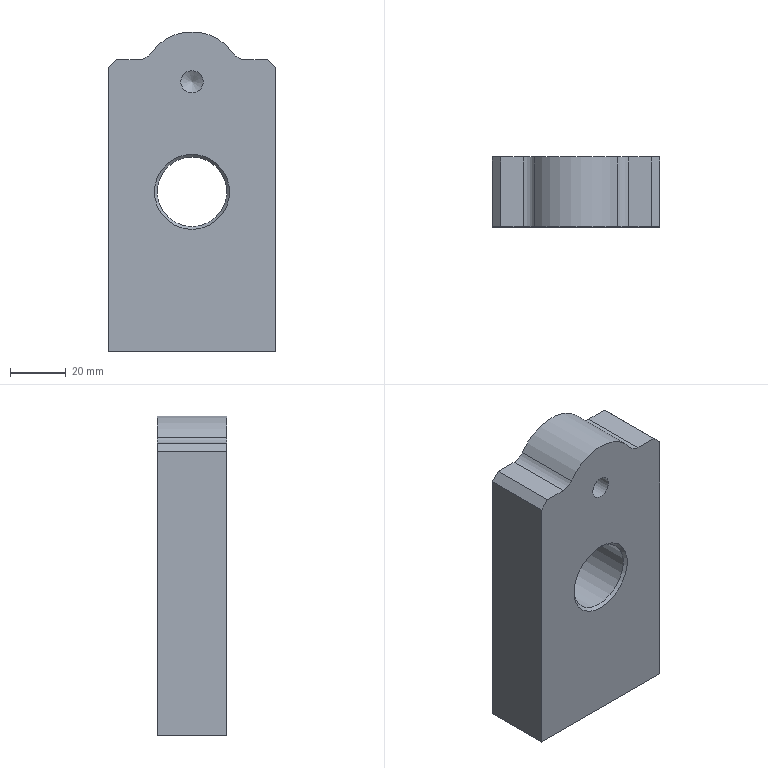Component | NX | 8_PILLAR | 1 solid | 21 faces | volume 148991 mm3 | plane 9 | cylinder 7 | cone 5 | commonest cylinder face diameters 10 x2 6 x2 36 x1 25 x1 8 x1